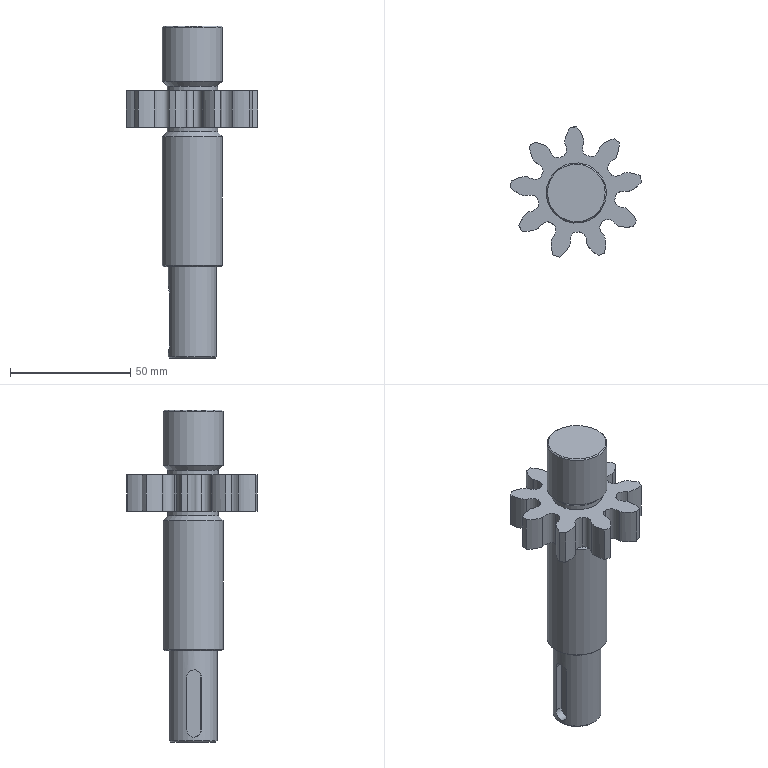Component | NX | CLYB_07_INPUTGEARSHAFT | 1 solid | 65 faces | volume 74746 mm3 | spline 36 | other 9 | plane 8 | cylinder 7 | cone 5 | commonest cylinder face diameters 21 x2 25 x2 6 x2 20 x1